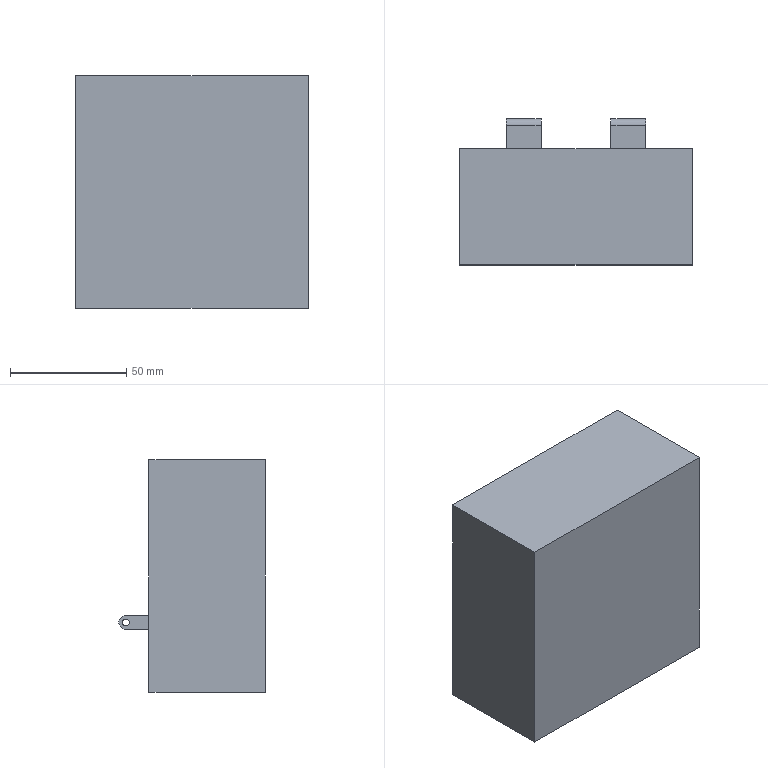Component | NX | PART_1 | 1 solid | 18 faces | volume 502012 mm3 | plane 14 | cylinder 4 | commonest cylinder face diameters 6 x2 3 x2